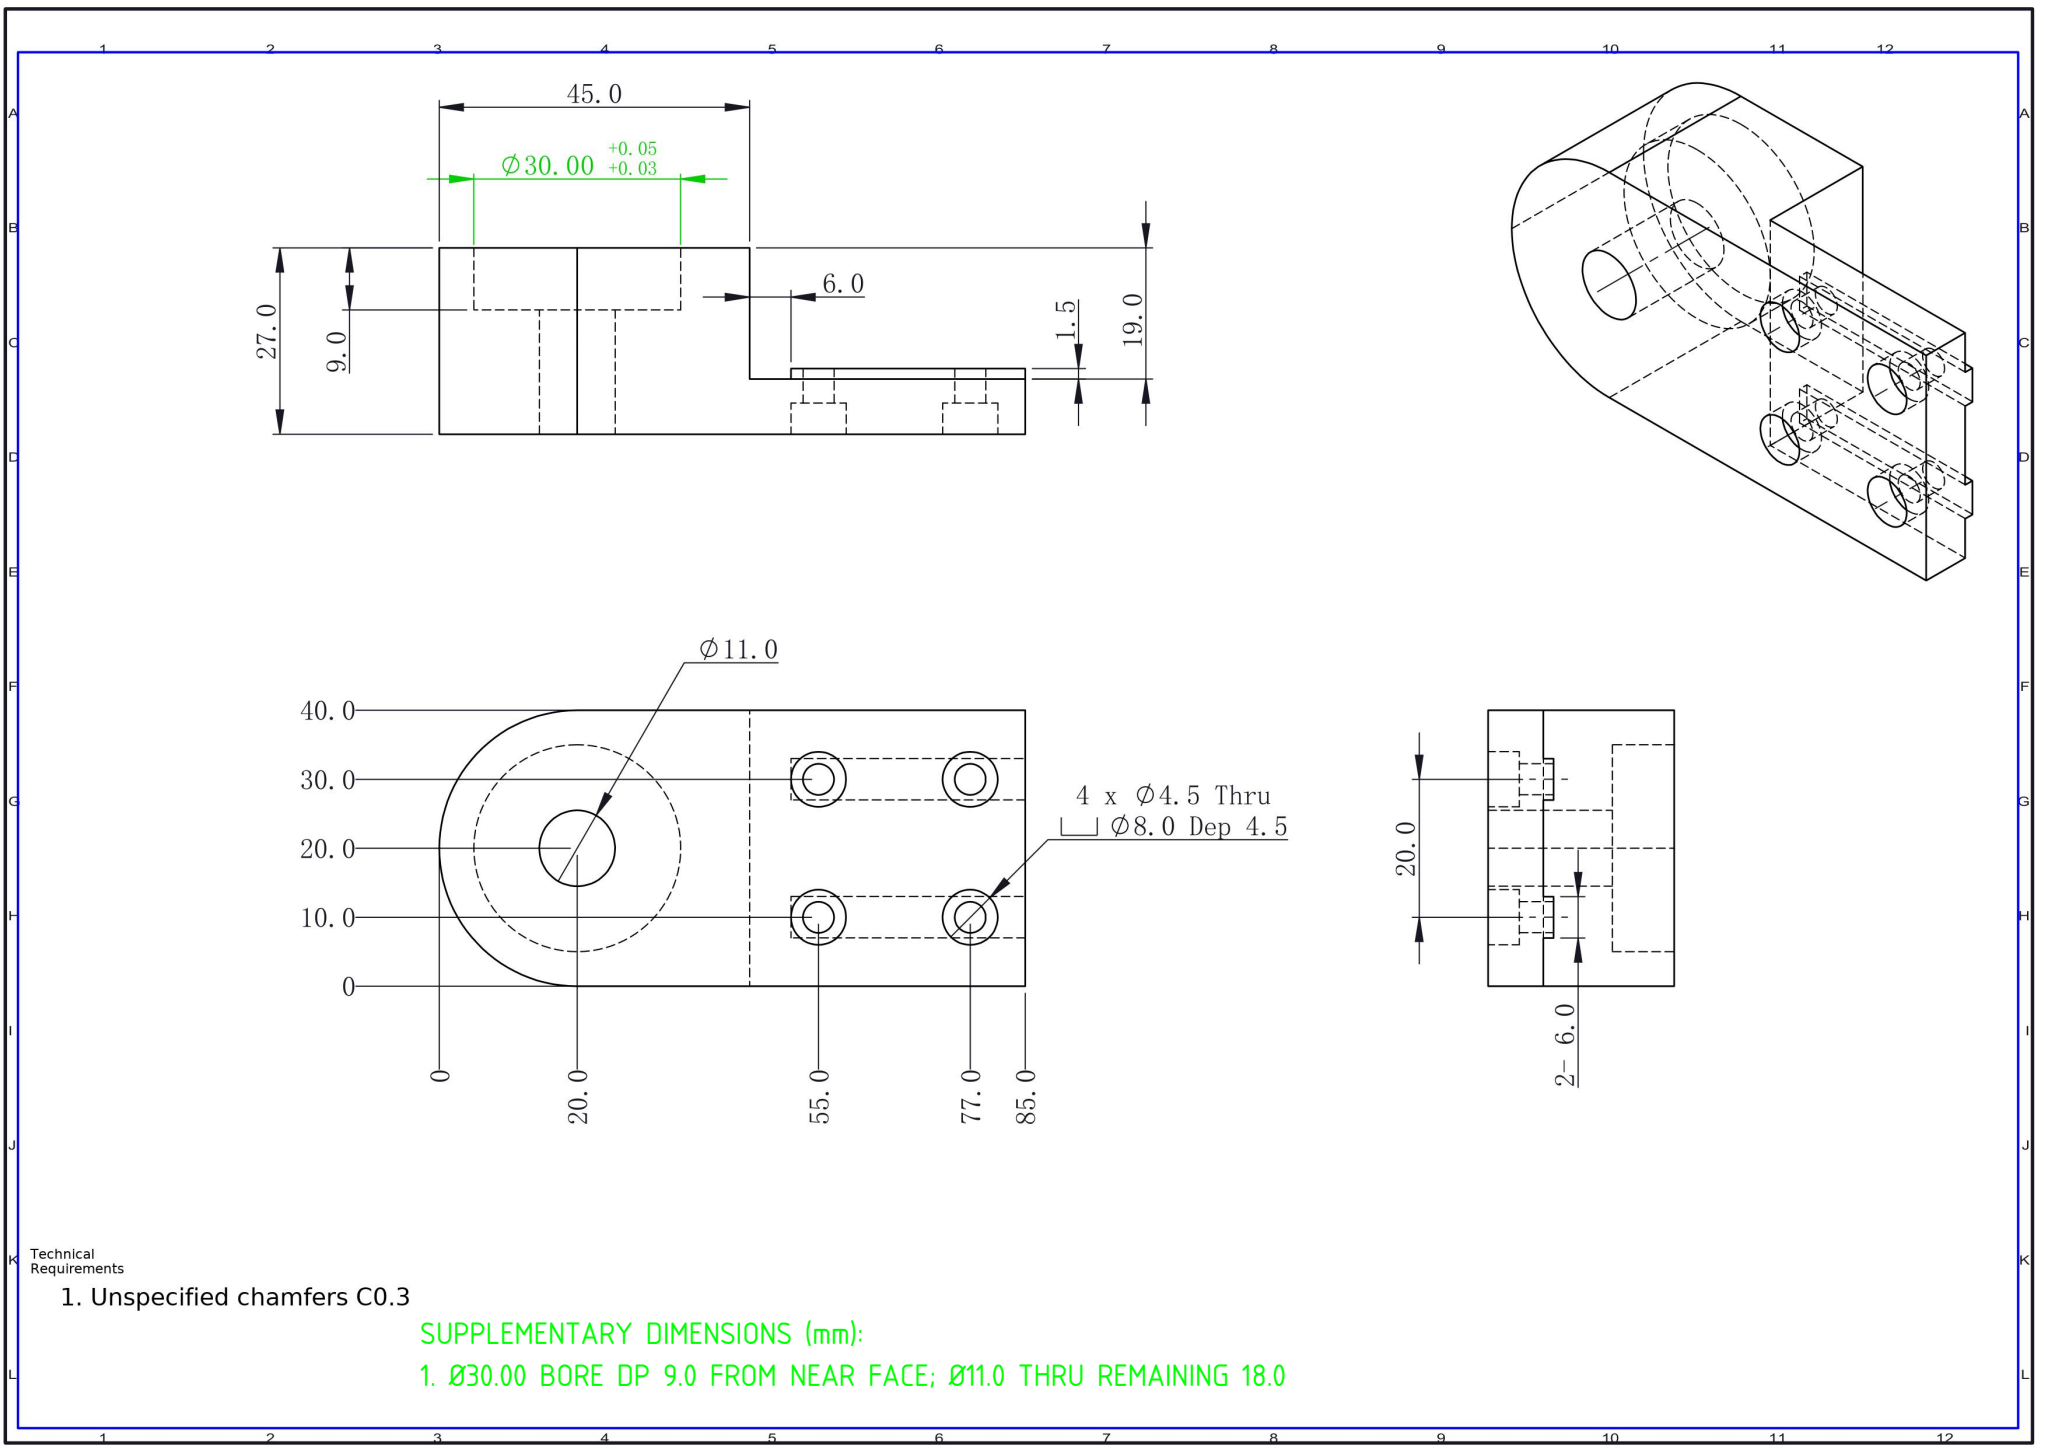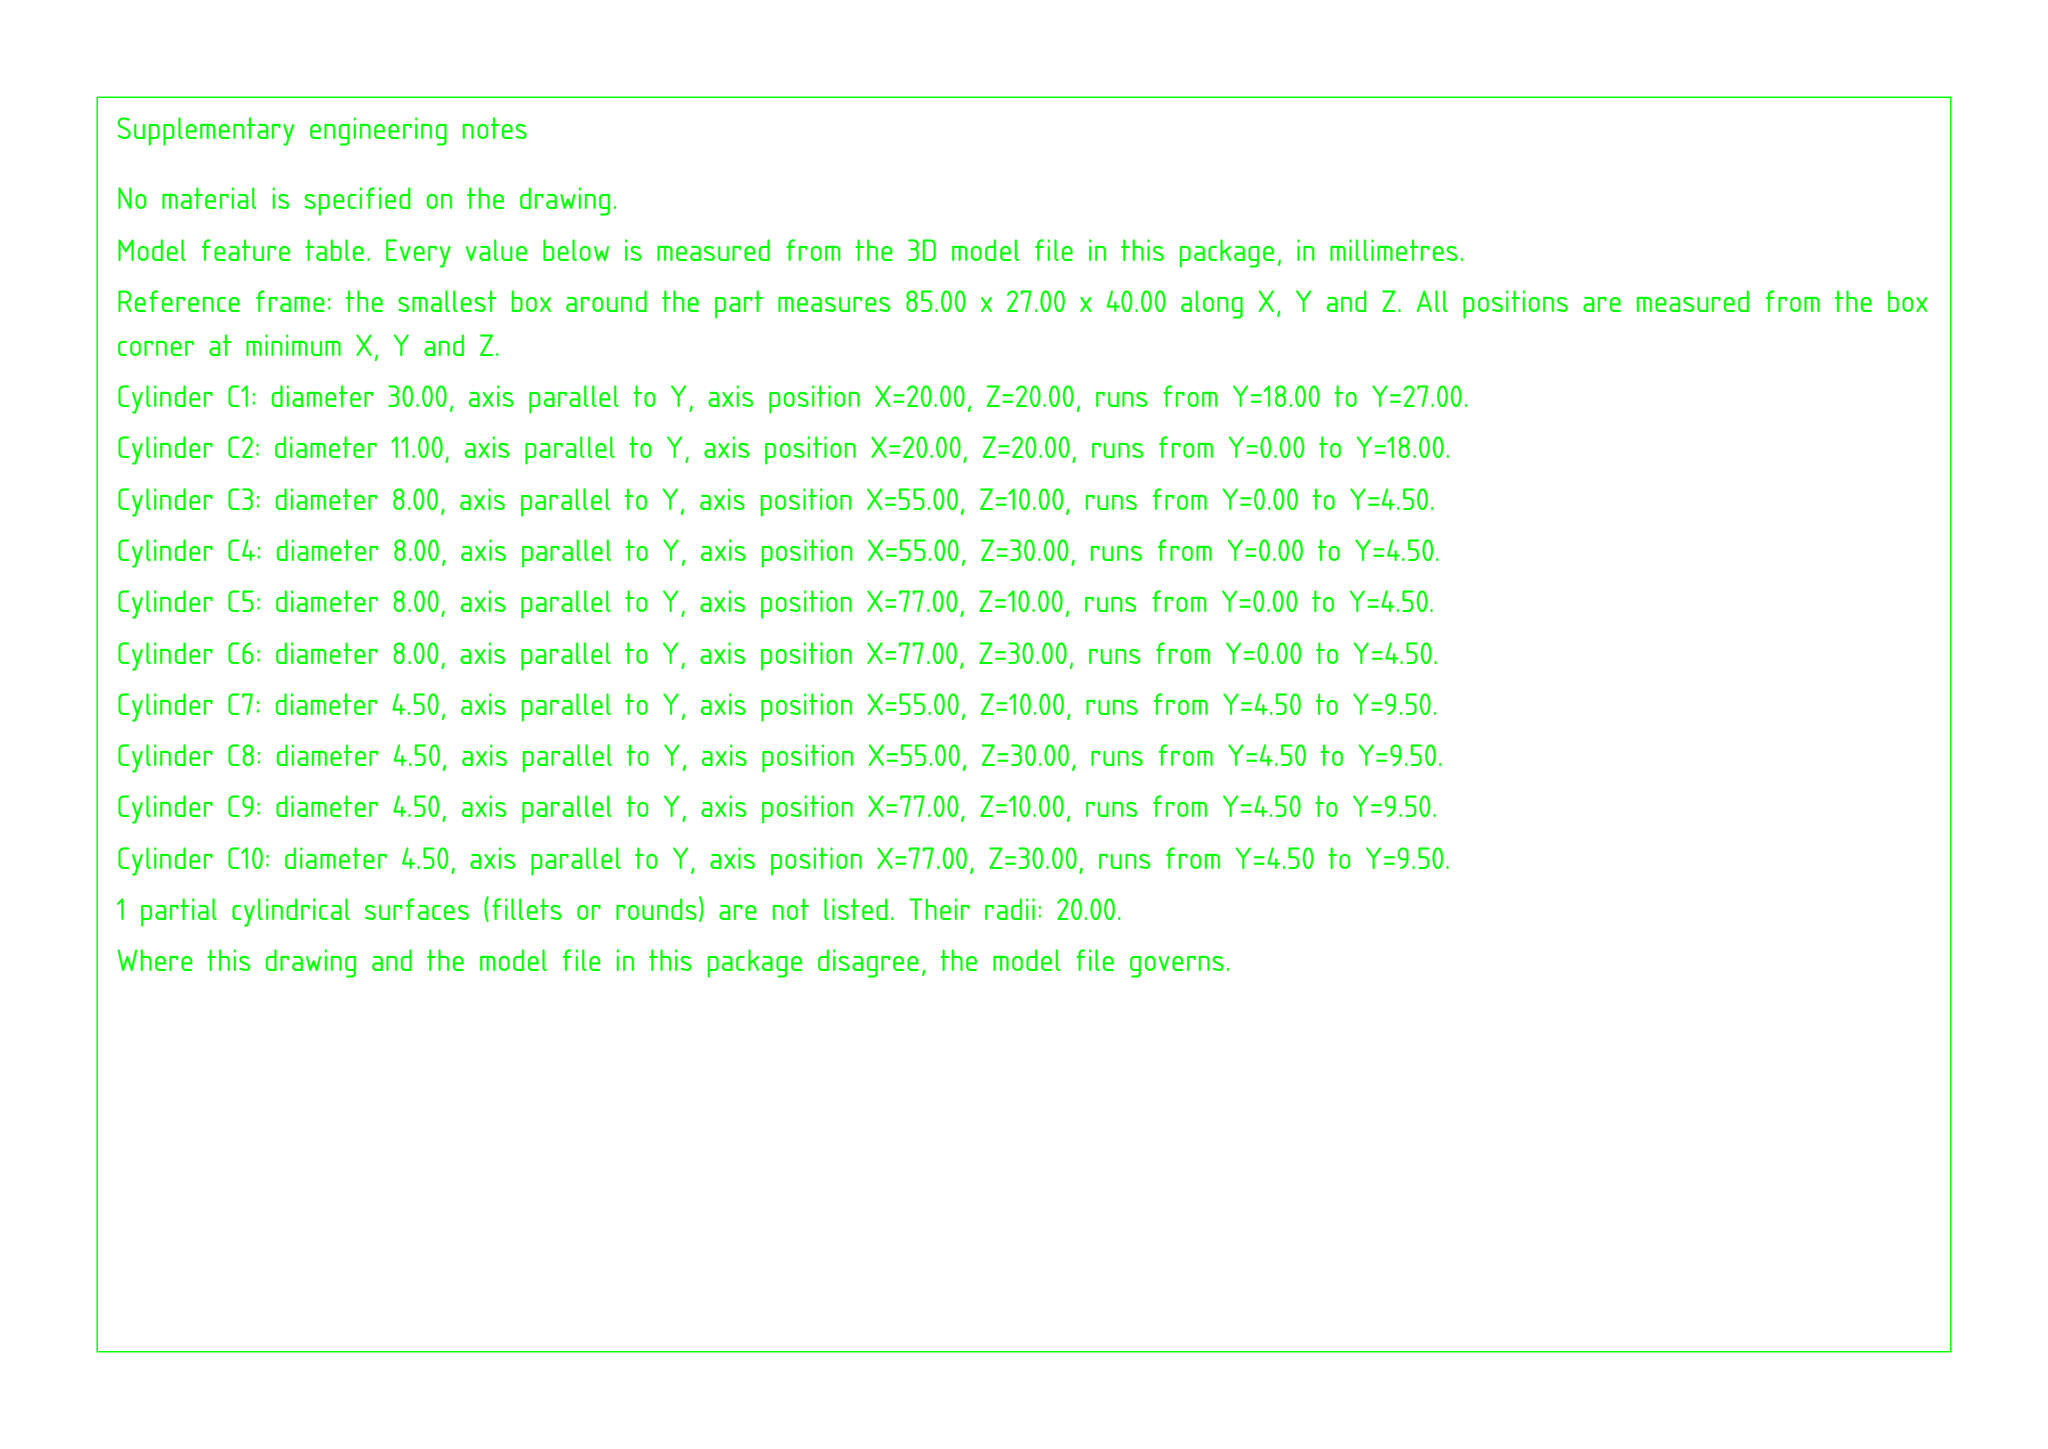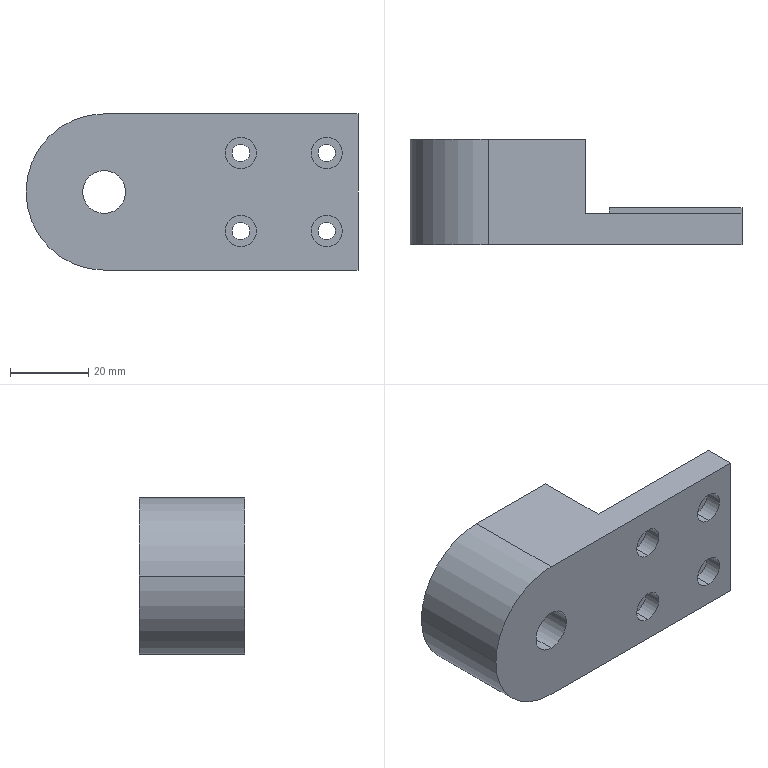Part | SolidWorks | mm | 1 solid | 42 faces | box 85 x 27 x 40 mm | volume 48081 mm3 | cylinder 22 | plane 20 | commonest cylinder face diameters 8 x8 4.5 x8 30 x2 11 x2 40 x2